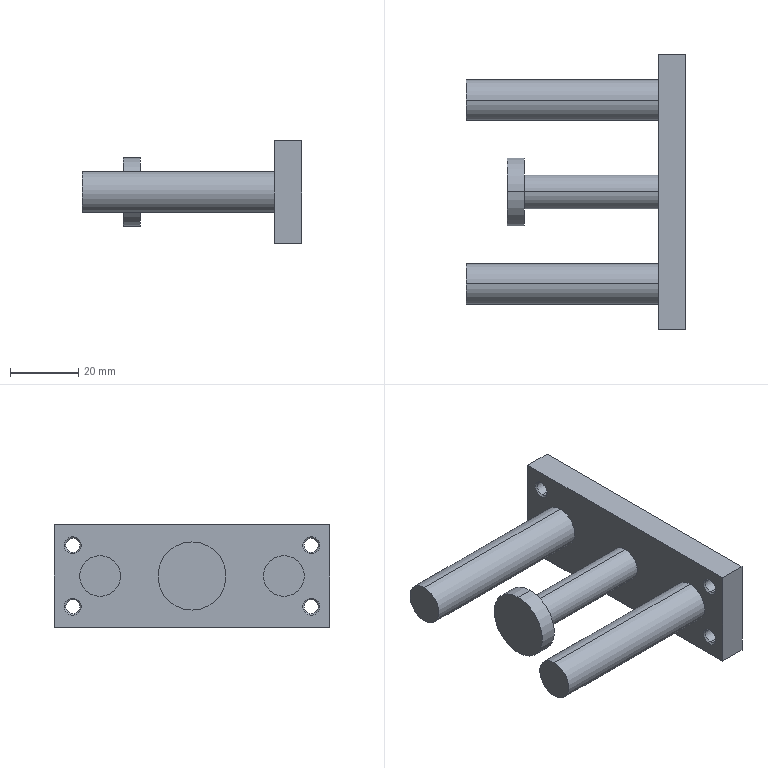Component | SolidWorks | MGPM20-20Z-M9P-1_MGPM20_20Z_0_ROD_4-1 | 1 solid | 56 faces | volume 36360 mm3 | cylinder 22 | cone 20 | plane 14 | commonest cylinder face diameters 4.134 x8 3 x6 12 x4 10 x2 20 x2